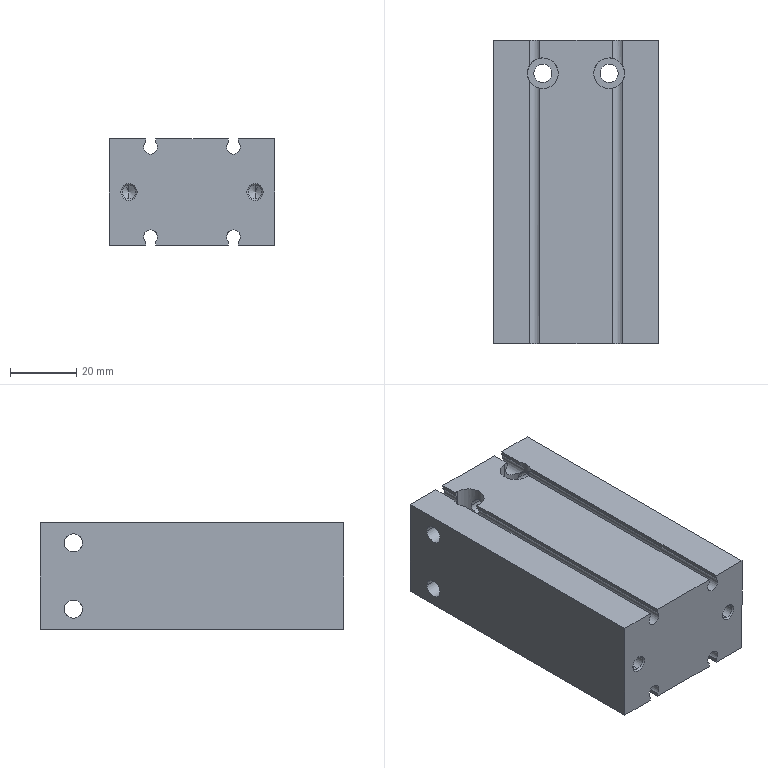Component | SolidWorks | HandlingMechanism-2_CDU25-40A-A93(0_0)-2_1.0.009603-1 | 1 solid | 114 faces | volume 111465 mm3 | cylinder 56 | plane 34 | cone 24 | commonest cylinder face diameters 5.5 x16 4.2 x12 4.134 x12 9.3 x8 10 x6 25 x2